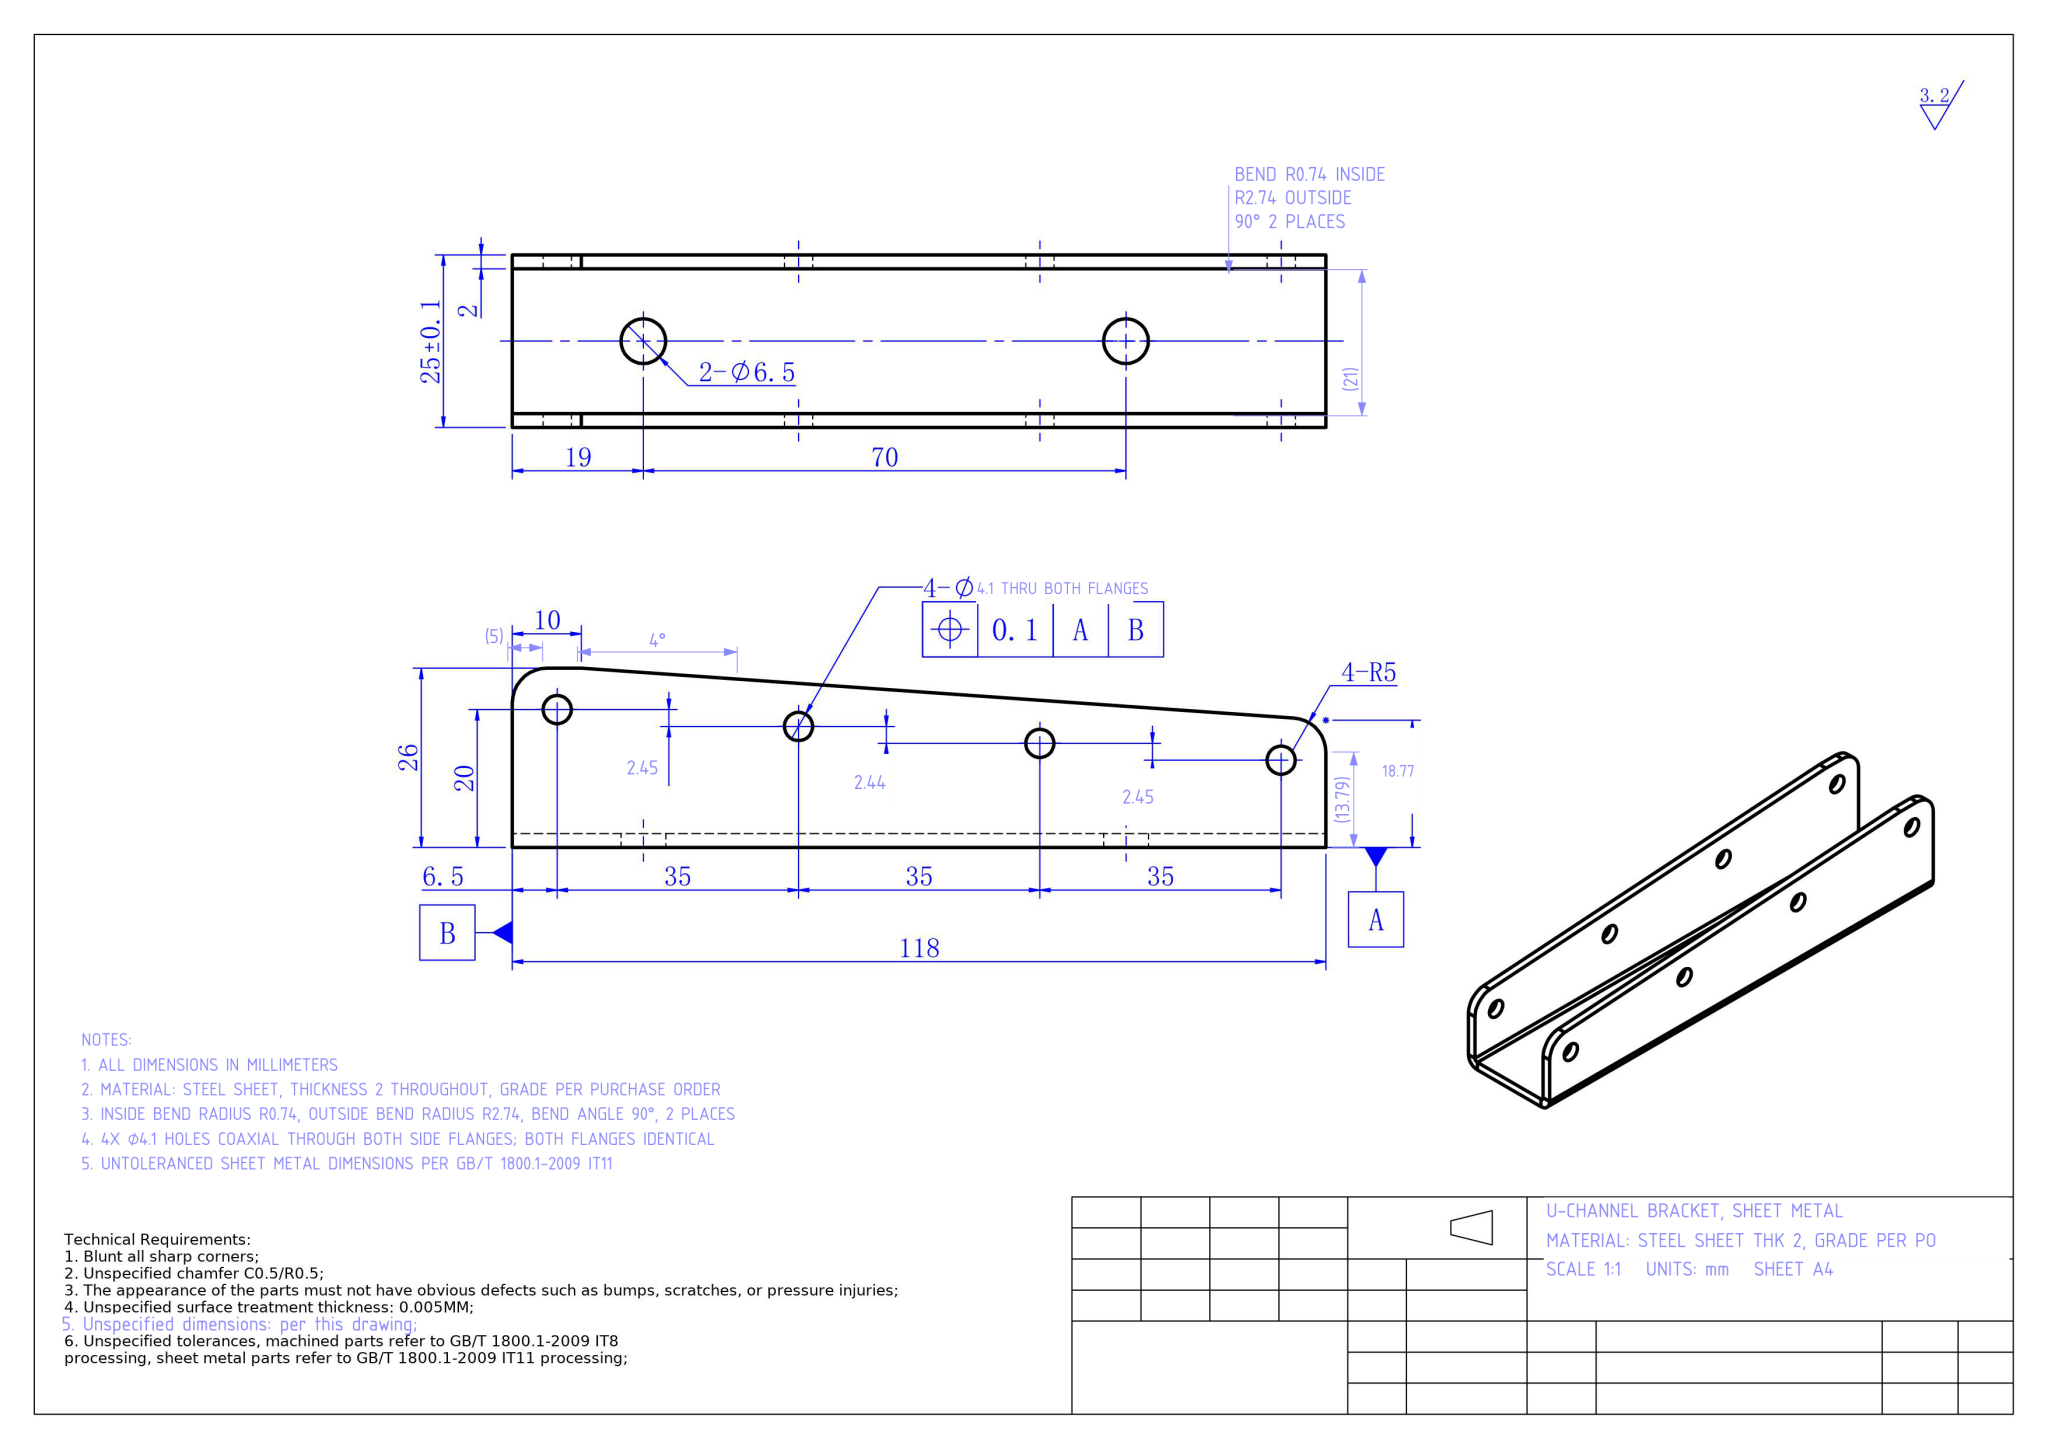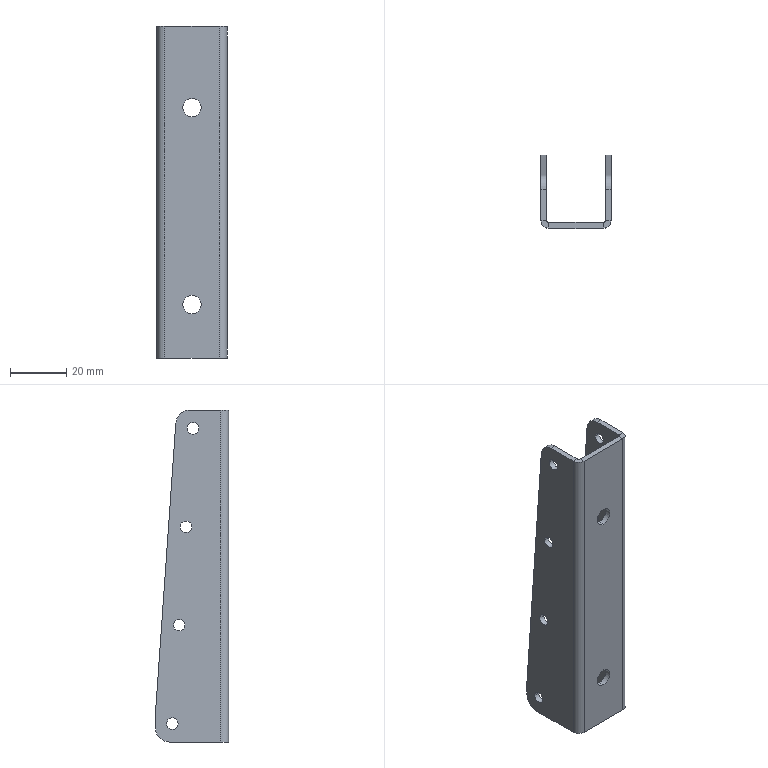Part | NX | mm | 1 solid | 48 faces | box 25 x 26 x 118 mm | volume 14861 mm3 | cylinder 28 | plane 20 | commonest cylinder face diameters 4.1 x16 6.5 x4 10 x4 1.473 x2 5.473 x2